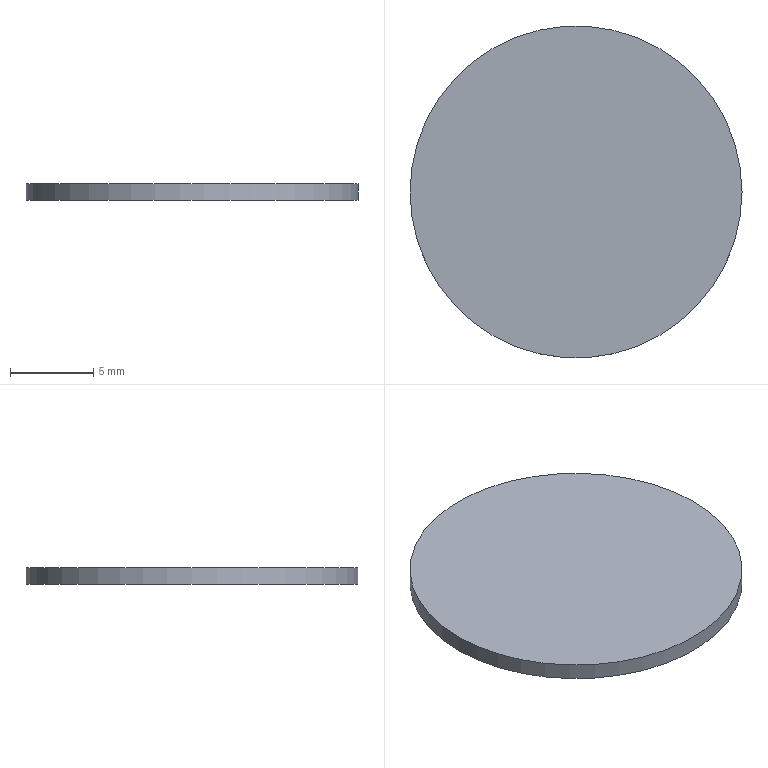Component | NX | DAMPING_PAD_2 | 1 solid | 3 faces | box 20 x 20 x 1 mm | volume 314 mm3 | plane 2 | cylinder 1 | commonest cylinder face diameters 20 x1
STEP:
#1=CARTESIAN_POINT('',(0.,0.,0.));
#2=DIRECTION('',(0.,0.,1.));
#3=DIRECTION('',(1.,0.,0.));
#4=AXIS2_PLACEMENT_3D('',#1,#2,#3);
#5=CARTESIAN_POINT('',(1.452,-94.62,-12.5));
#6=VERTEX_POINT('',#5);
#7=CARTESIAN_POINT('',(-8.548,-94.62,-12.5));
#8=DIRECTION('',(0.,0.,1.));
#9=DIRECTION('',(1.,0.,0.));
#10=AXIS2_PLACEMENT_3D('',#7,#8,#9);
#11=CIRCLE('',#10,10.);
#12=CARTESIAN_POINT('',(-8.548,-94.62,-12.5));
#13=DIRECTION('',(0.,0.,-1.));
#14=DIRECTION('',(-1.,0.,0.));
#15=AXIS2_PLACEMENT_3D('',#12,#13,#14);
#16=CYLINDRICAL_SURFACE('',#15,10.);
#17=CARTESIAN_POINT('',(9.425,0.));
#18=DIRECTION('',(-1.,0.));
#19=VECTOR('',#18,1.);
#20=LINE('',#17,#19);
#21=(GEOMETRIC_REPRESENTATION_CONTEXT(2)PARAMETRIC_REPRESENTATION_CONTEXT()REPRESENTATION_CONTEXT('',''));
#22=DEFINITIONAL_REPRESENTATION('',(#20),#21);
#23=PCURVE('',#16,#22);
#24=CARTESIAN_POINT('',(-8.548,-94.62,-12.5));
#25=DIRECTION('',(0.,0.,1.));
#26=DIRECTION('',(1.,0.,0.));
#27=AXIS2_PLACEMENT_3D('',#24,#25,#26);
#28=PLANE('',#27);
#29=CARTESIAN_POINT('',(0.,0.));
#30=DIRECTION('',(1.,0.));
#31=AXIS2_PLACEMENT_2D('',#29,#30);
#32=CIRCLE('',#31,10.);
#33=(GEOMETRIC_REPRESENTATION_CONTEXT(2)PARAMETRIC_REPRESENTATION_CONTEXT()REPRESENTATION_CONTEXT('',''));
#34=DEFINITIONAL_REPRESENTATION('',(#32),#33);
#35=PCURVE('',#28,#34);
#36=SURFACE_CURVE('',#11,(#23,#35),.PCURVE_S1.);
#37=EDGE_CURVE('',#6,#6,#36,.T.);
#38=ORIENTED_EDGE('',*,*,#37,.F.);
#39=CARTESIAN_POINT('',(1.452,-94.62,-13.5));
#40=VERTEX_POINT('',#39);
#41=CARTESIAN_POINT('',(1.452,-94.62,-12.5));
#42=CARTESIAN_POINT('',(1.452,-94.62,-13.5));
#43=B_SPLINE_CURVE_WITH_KNOTS('',1,(#41,#42),.UNSPECIFIED.,.F.,.F.,(2,2),(0.,1.),.PIECEWISE_BEZIER_KNOTS.);
#44=CARTESIAN_POINT('',(9.425,0.));
#45=DIRECTION('',(0.,1.));
#46=VECTOR('',#45,1.);
#47=LINE('',#44,#46);
#48=(GEOMETRIC_REPRESENTATION_CONTEXT(2)PARAMETRIC_REPRESENTATION_CONTEXT()REPRESENTATION_CONTEXT('',''));
#49=DEFINITIONAL_REPRESENTATION('',(#47),#48);
#50=PCURVE('',#16,#49);
#51=CARTESIAN_POINT('',(3.142,0.));
#52=DIRECTION('',(0.,1.));
#53=VECTOR('',#52,1.);
#54=LINE('',#51,#53);
#55=(GEOMETRIC_REPRESENTATION_CONTEXT(2)PARAMETRIC_REPRESENTATION_CONTEXT()REPRESENTATION_CONTEXT('',''));
#56=DEFINITIONAL_REPRESENTATION('',(#54),#55);
#57=PCURVE('',#16,#56);
#58=SEAM_CURVE('',#43,(#50,#57),.PCURVE_S1.);
#59=EDGE_CURVE('',#6,#40,#58,.T.);
#60=ORIENTED_EDGE('',*,*,#59,.T.);
#61=CARTESIAN_POINT('',(-8.548,-94.62,-13.5));
#62=DIRECTION('',(0.,0.,1.));
#63=DIRECTION('',(1.,0.,0.));
#64=AXIS2_PLACEMENT_3D('',#61,#62,#63);
#65=CIRCLE('',#64,10.);
#66=CARTESIAN_POINT('',(9.425,1.));
#67=DIRECTION('',(-1.,0.));
#68=VECTOR('',#67,1.);
#69=LINE('',#66,#68);
#70=(GEOMETRIC_REPRESENTATION_CONTEXT(2)PARAMETRIC_REPRESENTATION_CONTEXT()REPRESENTATION_CONTEXT('',''));
#71=DEFINITIONAL_REPRESENTATION('',(#69),#70);
#72=PCURVE('',#16,#71);
#73=CARTESIAN_POINT('',(-8.548,-94.62,-13.5));
#74=DIRECTION('',(0.,0.,1.));
#75=DIRECTION('',(1.,0.,0.));
#76=AXIS2_PLACEMENT_3D('',#73,#74,#75);
#77=PLANE('',#76);
#78=CARTESIAN_POINT('',(0.,0.));
#79=DIRECTION('',(1.,0.));
#80=AXIS2_PLACEMENT_2D('',#78,#79);
#81=CIRCLE('',#80,10.);
#82=(GEOMETRIC_REPRESENTATION_CONTEXT(2)PARAMETRIC_REPRESENTATION_CONTEXT()REPRESENTATION_CONTEXT('',''));
#83=DEFINITIONAL_REPRESENTATION('',(#81),#82);
#84=PCURVE('',#77,#83);
#85=SURFACE_CURVE('',#65,(#72,#84),.PCURVE_S1.);
#86=EDGE_CURVE('',#40,#40,#85,.T.);
#87=ORIENTED_EDGE('',*,*,#86,.T.);
#88=ORIENTED_EDGE('',*,*,#59,.F.);
#89=EDGE_LOOP('',(#38,#60,#87,#88));
#90=FACE_BOUND('',#89,.T.);
#91=ADVANCED_FACE('',(#90),#16,.T.);
#92=ORIENTED_EDGE('',*,*,#37,.T.);
#93=EDGE_LOOP('',(#92));
#94=FACE_BOUND('',#93,.T.);
#95=ADVANCED_FACE('',(#94),#28,.T.);
#96=ORIENTED_EDGE('',*,*,#86,.F.);
#97=EDGE_LOOP('',(#96));
#98=FACE_BOUND('',#97,.T.);
#99=ADVANCED_FACE('',(#98),#77,.F.);
#100=CLOSED_SHELL('',(#91,#95,#99));
#101=MANIFOLD_SOLID_BREP('',#100);
#102=(LENGTH_UNIT()NAMED_UNIT(*)SI_UNIT(.MILLI.,.METRE.));
#103=UNCERTAINTY_MEASURE_WITH_UNIT(LENGTH_MEASURE(0.00001),#102,'','');
#104=(NAMED_UNIT(*)PLANE_ANGLE_UNIT()SI_UNIT($,.RADIAN.));
#105=(NAMED_UNIT(*)SI_UNIT($,.STERADIAN.)SOLID_ANGLE_UNIT());
#106=(GEOMETRIC_REPRESENTATION_CONTEXT(3)GLOBAL_UNCERTAINTY_ASSIGNED_CONTEXT((#103))GLOBAL_UNIT_ASSIGNED_CONTEXT((#102,#104,#105))REPRESENTATION_CONTEXT('',''));
#107=ADVANCED_BREP_SHAPE_REPRESENTATION('',(#4,#101),#106);